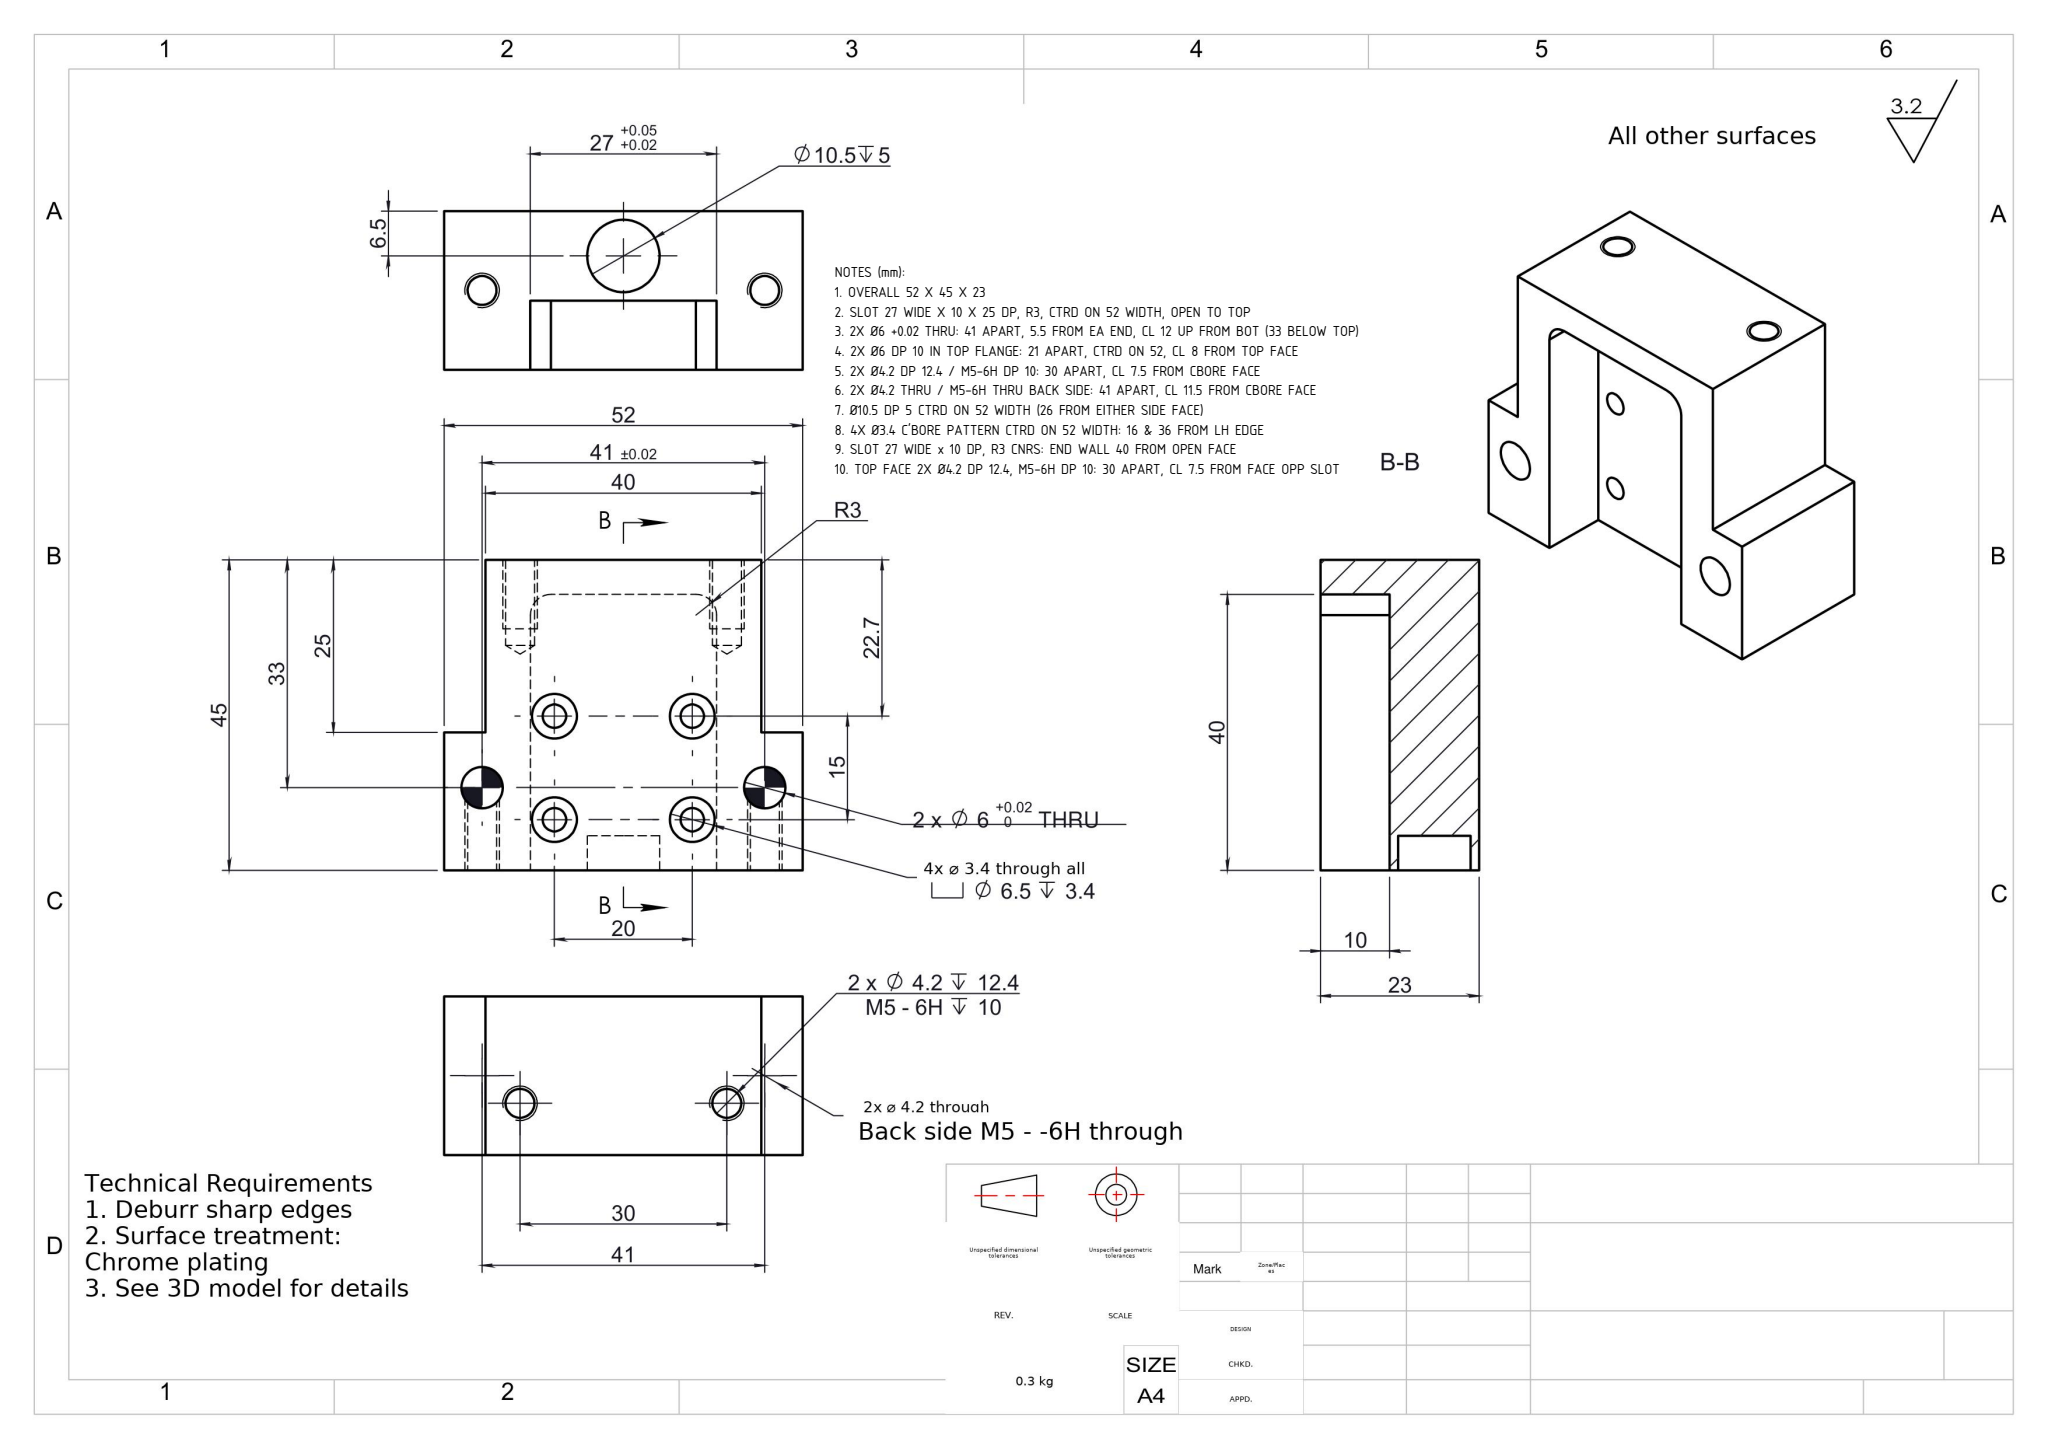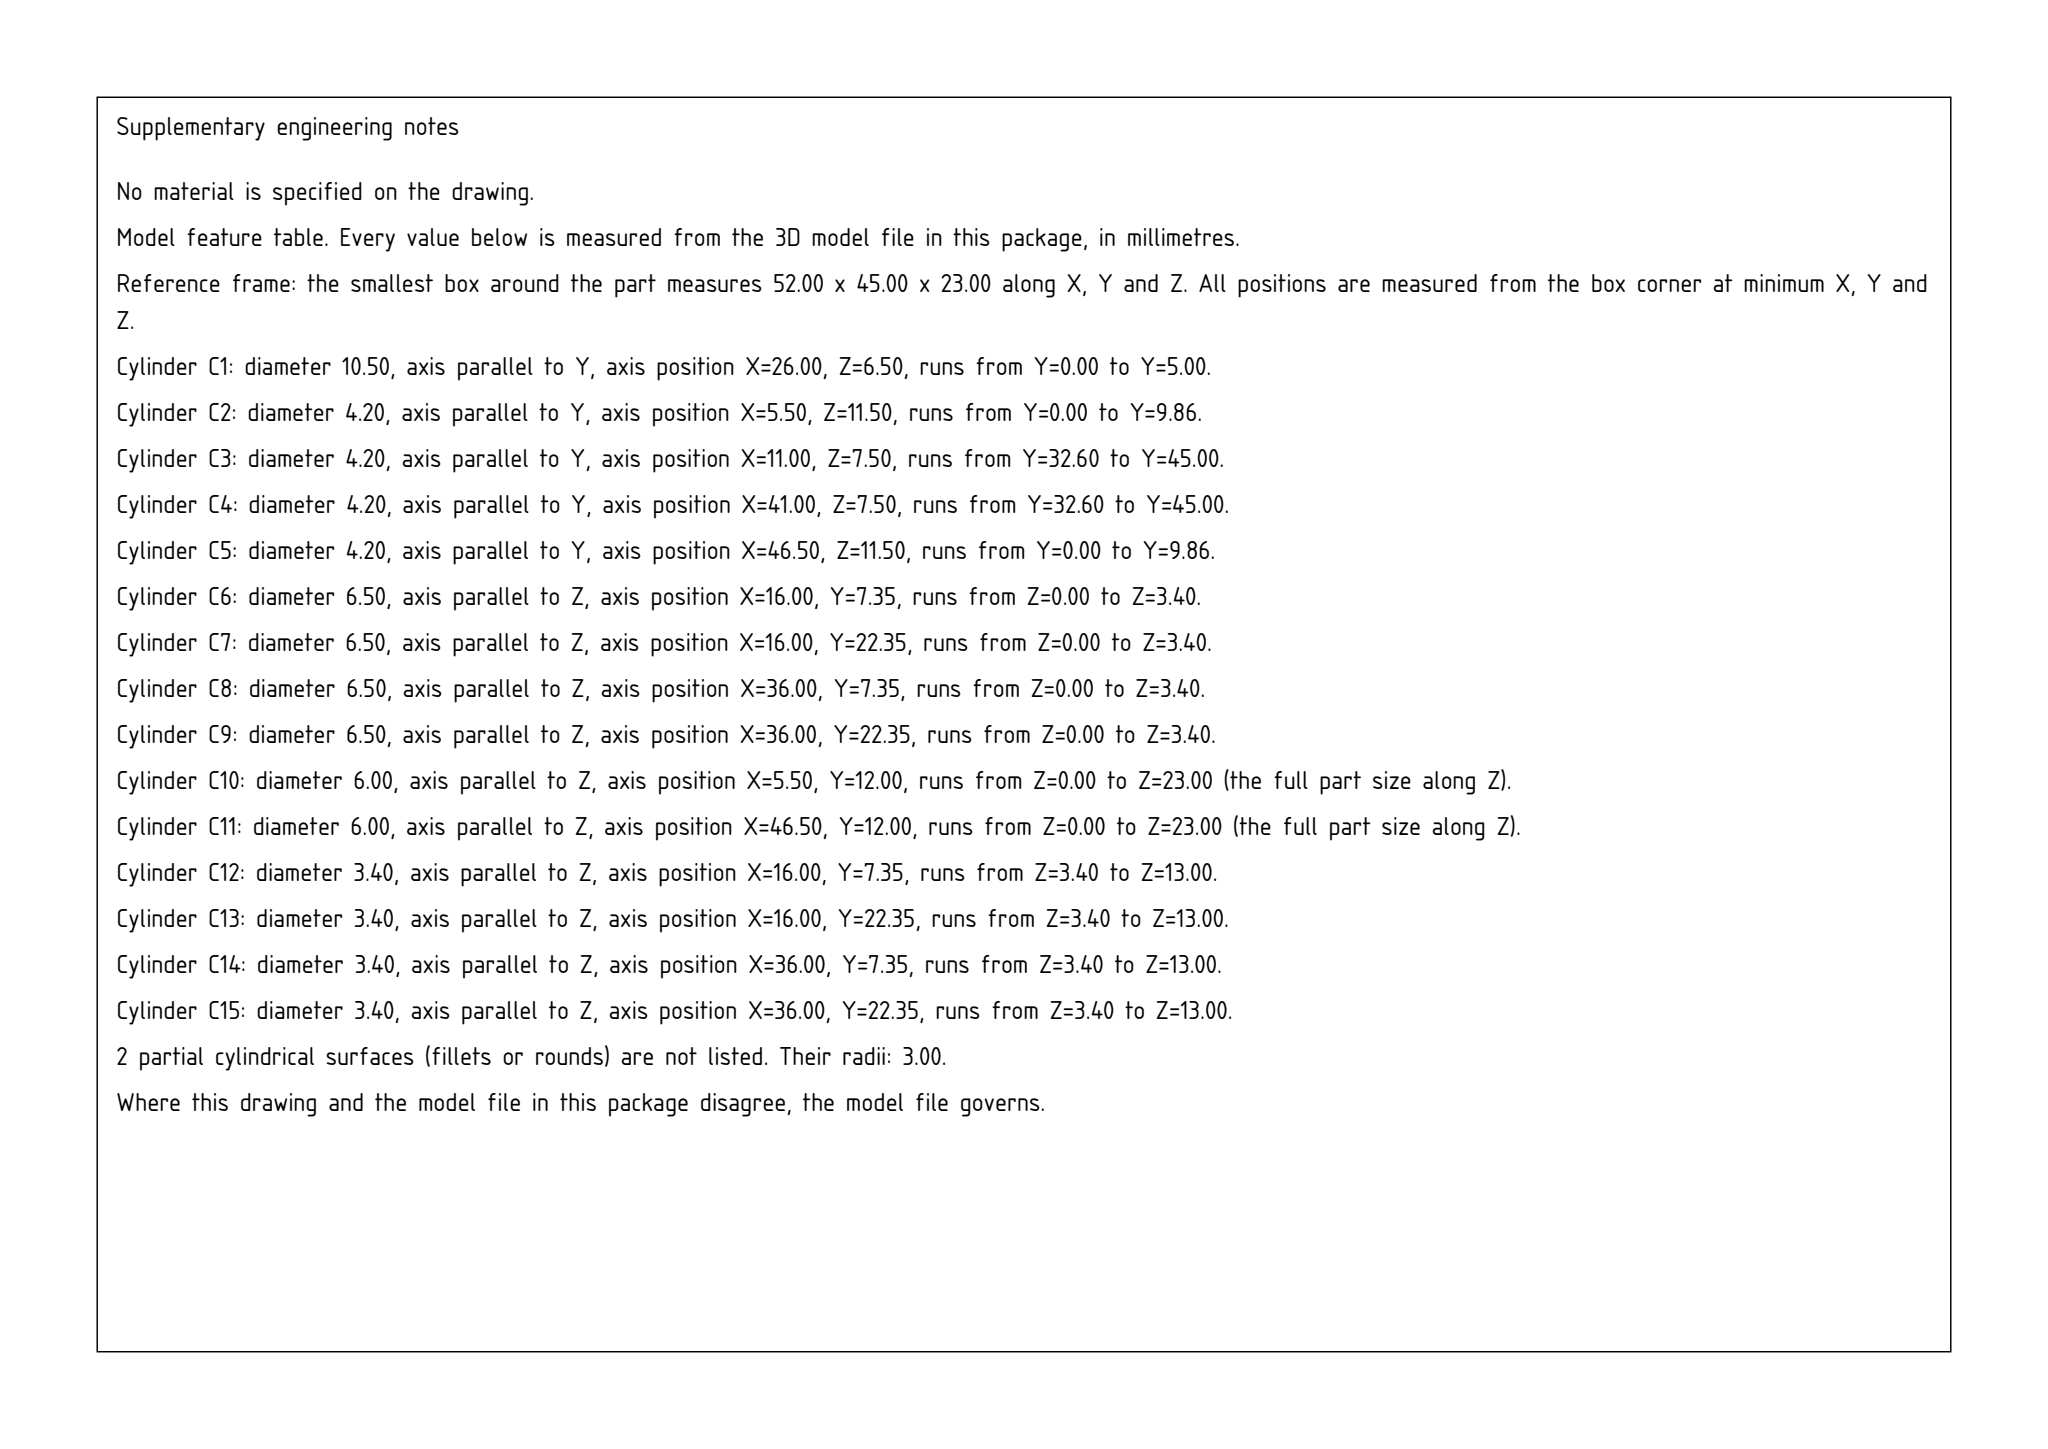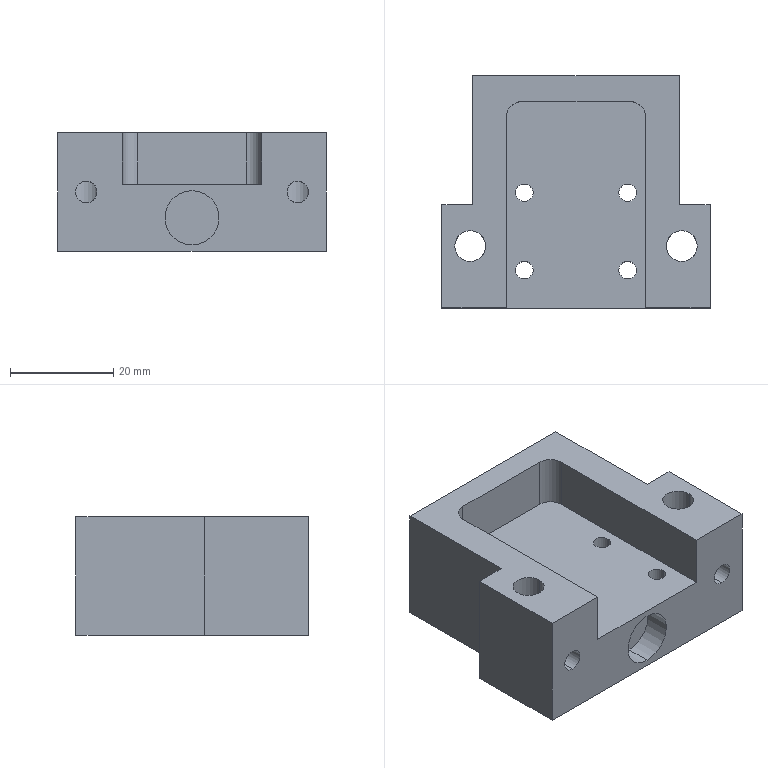Part | SolidWorks | mm | 1 solid | 55 faces | box 52 x 45 x 23 mm | volume 33015 mm3 | cylinder 32 | plane 19 | cone 4 | commonest cylinder face diameters 4.2 x8 6.5 x8 3.4 x8 6 x6 10.5 x2
Drawing notes:
OVERALL 52 X 45 X 23 | from the solid: bbox_xyz [52.0, 45.0, 23.0]
SLOT 27 WIDE X 10 X 25 DP, R3, CTRD ON 52 WIDTH, OPEN TO TOP | from the solid: x-planes 12.5 & 39.5 = 27 wide, ctr 26 = 52/2; z-plane 13 to z=23 face = 10; y-plane 20 to y=45 top = 25 dp
2X Ø6 +0.02 THRU: 41 APART, 5.5 FROM EA END, CL 12 UP FROM BOT (33 BELOW TOP) | from the solid: Ø6 z-axis cyls at (x5.5,y12) & (x46.5,y12), len 23 = full thk; 46.5-5.5=41; 52-46.5=5.5; 45-12=33
2X Ø6 DP 10 IN TOP FLANGE: 21 APART, CTRD ON 52, CL 8 FROM TOP FACE | from the solid: Ø6 z-axis cyls at (x15.5,y37) & (x36.5,y37), len 10 (z13 to z23); 36.5-15.5=21, ctr 26 = 52/2; 45-37=8
2X Ø4.2 DP 12.4 / M5-6H DP 10: 30 APART, CL 7.5 FROM CBORE FACE | from the solid: Ø4.2 y-axis cyls at (x11,z7.5) & (x41,z7.5), len 12.4 with 118° point; 41-11=30; z=7.5 from z=0 face carrying Ø6.5 cbores
2X Ø4.2 THRU / M5-6H THRU BACK SIDE: 41 APART, CL 11.5 FROM CBORE FACE | from the solid: Ø4.2 y-axis cyls at (x5.5,z11.5) & (x46.5,z11.5), len 9.86, no cone = thru into Ø6 holes; 46.5-5.5=41; z=11.5 = 23/2
Ø10.5 DP 5 CTRD ON 52 WIDTH (26 FROM EITHER SIDE FACE) | from the solid: hole/bore dia 10.5 axis y at x=26.0, bbox x extent 0-52 -> centred
4X Ø3.4 C'BORE PATTERN CTRD ON 52 WIDTH: 16 & 36 FROM LH EDGE | from the solid: Ø3.4/Ø6.5 holes at x=16.0 and x=36.0, bbox x 0-52; 20 apart, symmetric about 26
SLOT 27 WIDE x 10 DP, R3 CNRS: END WALL 40 FROM OPEN FACE | from the solid: Floor plane z=13 x[12.5,39.5] y[0,40] (27 wide, 23-13=10 dp); end wall plane y=40 x[15.5,36.5] z[13,23]; R3 arcs dia 6 at (15.5,37) and (36.5,37)
TOP FACE 2X Ø4.2 DP 12.4, M5-6H DP 10: 30 APART, CL 7.5 FROM FACE OPP SLOT | from the solid: Ø4.2 y-axis holes at x=11 and x=41, z=7.5, from y=32.6 to y=45 (12.4 deep from top face y=45); 41-11=30 apart, ctrd on 52; slot opens at z=23
build123d program:
from build123d import *

# Parameters (mm, degrees)
SKETCH1_W                                       = 52
SKETCH1_H                                       = 45
BOSS_EXTRUDE1_DEPTH                             = 23
SKETCH2_W                                       = 27
SKETCH2_H                                       = 40
CUT_EXTRUDE1_DEPTH                              = 10
SKETCH3_R                                       = 5.25
CUT_EXTRUDE2_DEPTH                              = 5
SKETCH4_W                                       = 6
SKETCH4_H                                       = 25
CUT_EXTRUDE3_DEPTH                              = 42.367
SIZE_MM_DOWEL_HOLE_1_D                          = 6
FILLET1_R                                       = 3
M5_TAPPED_HOLE1_D                               = 4.2
M5_TAPPED_HOLE1_DEPTH                           = 12.4
M5_TAPPED_HOLE1_TIP                             = 1.262
M3_HEX_SOCKET_HEAD_CAP_SCREW_CBORE1_D           = 3.4
M3_HEX_SOCKET_HEAD_CAP_SCREW_CBORE1_CBORE_D     = 6.5
M3_HEX_SOCKET_HEAD_CAP_SCREW_CBORE1_CBORE_DEPTH = 3.4
M5_TAPPED_HOLE2_REACH                           = 58.833
M5_TAPPED_HOLE2_BORE_R                          = 2.1


with BuildPart() as part:
    # Sketch1 → Boss-Extrude1 (new body)
    with BuildSketch(Plane.XY):
        Rectangle(SKETCH1_W, SKETCH1_H)
    extrude(amount=BOSS_EXTRUDE1_DEPTH)

    # Sketch2 → Cut-Extrude1 (cut)
    with BuildSketch(Plane.XY.offset(23)):
        with Locations((0, -2.5)):
            Rectangle(SKETCH2_W, SKETCH2_H)
    extrude(amount=-CUT_EXTRUDE1_DEPTH, mode=Mode.SUBTRACT)

    # Sketch3 → Cut-Extrude2 (cut)
    with BuildSketch(Plane.XZ.offset(22.5)):
        with Locations(Location((0, 6.5, 0), (0, 0, 270))):
            Circle(SKETCH3_R)
    extrude(amount=-CUT_EXTRUDE2_DEPTH, mode=Mode.SUBTRACT)

    # Sketch4 → Cut-Extrude3 (cut, through all)
    with BuildSketch(Plane(origin=(0, 0, 0), x_dir=(-1, 0, 0), z_dir=(0, 0, -1))):
        with Locations((-23, 10)):
            Rectangle(SKETCH4_W, SKETCH4_H)
        with Locations((23, 10)):
            Rectangle(SKETCH4_W, SKETCH4_H)
    extrude(amount=-CUT_EXTRUDE3_DEPTH, mode=Mode.SUBTRACT)

    # Size mm Dowel Hole 1 (through all)
    with Locations(Plane(origin=(0, 0, 0), x_dir=(-1, 0, 0), z_dir=(0, 0, -1))):
        with Locations((-20.5, -10.5), (20.5, -10.5)):
            Hole(SIZE_MM_DOWEL_HOLE_1_D / 2)

    # Fillet1
    fillet1_edges = [part.edges().sort_by_distance(p)[0] for p in [
        (-13.5, 17.5, 18),
        (13.5, 17.5, 18),
    ]]
    fillet(fillet1_edges, radius=FILLET1_R)

    # M5 Tapped Hole1
    with Locations(Plane(origin=(0, 22.5, 0), x_dir=(1, 0, 0), z_dir=(0, 1, 0))):
        with Locations((15, -7.5), (-15, -7.5)):
            Hole(M5_TAPPED_HOLE1_D / 2, depth=M5_TAPPED_HOLE1_DEPTH)
            with Locations((0, 0, -(M5_TAPPED_HOLE1_DEPTH + M5_TAPPED_HOLE1_TIP / 2))):  # 118° drill point
                Cone(0, M5_TAPPED_HOLE1_D / 2, M5_TAPPED_HOLE1_TIP, mode=Mode.SUBTRACT)

    # M3 Hex Socket Head Cap Screw CBORE1 (through all)
    with Locations(Plane(origin=(0, 0, 0), x_dir=(-1, 0, 0), z_dir=(0, 0, -1))):
        with Locations((-10, -15.15), (-10, -0.15), (10, -0.15), (10, -15.15)):
            CounterBoreHole(M3_HEX_SOCKET_HEAD_CAP_SCREW_CBORE1_D / 2, M3_HEX_SOCKET_HEAD_CAP_SCREW_CBORE1_CBORE_D / 2, M3_HEX_SOCKET_HEAD_CAP_SCREW_CBORE1_CBORE_DEPTH)

    # M5 Tapped Hole2 bore → M5 Tapped Hole2 (cut, up to next)
    with BuildSketch(Plane.XZ.offset(22.5), mode=Mode.PRIVATE) as m5_tapped_hole2_sk1:
        with Locations((-20.5, 11.5)):
            Circle(M5_TAPPED_HOLE2_BORE_R)
    m5_tapped_hole2_tool1 = extrude(m5_tapped_hole2_sk1.sketch, amount=-M5_TAPPED_HOLE2_REACH, mode=Mode.PRIVATE) & part.part
    # M5 Tapped Hole2 bore → M5 Tapped Hole2 (cut, up to next)
    with BuildSketch(Plane.XZ.offset(22.5), mode=Mode.PRIVATE) as m5_tapped_hole2_sk2:
        with Locations((20.5, 11.5)):
            Circle(M5_TAPPED_HOLE2_BORE_R)
    m5_tapped_hole2_tool2 = extrude(m5_tapped_hole2_sk2.sketch, amount=-M5_TAPPED_HOLE2_REACH, mode=Mode.PRIVATE) & part.part
    add(m5_tapped_hole2_tool1.solids().sort_by_distance((-20.5, -22.5, 11.5))[0], mode=Mode.SUBTRACT)
    add(m5_tapped_hole2_tool2.solids().sort_by_distance((20.5, -22.5, 11.5))[0], mode=Mode.SUBTRACT)


solid = part.part